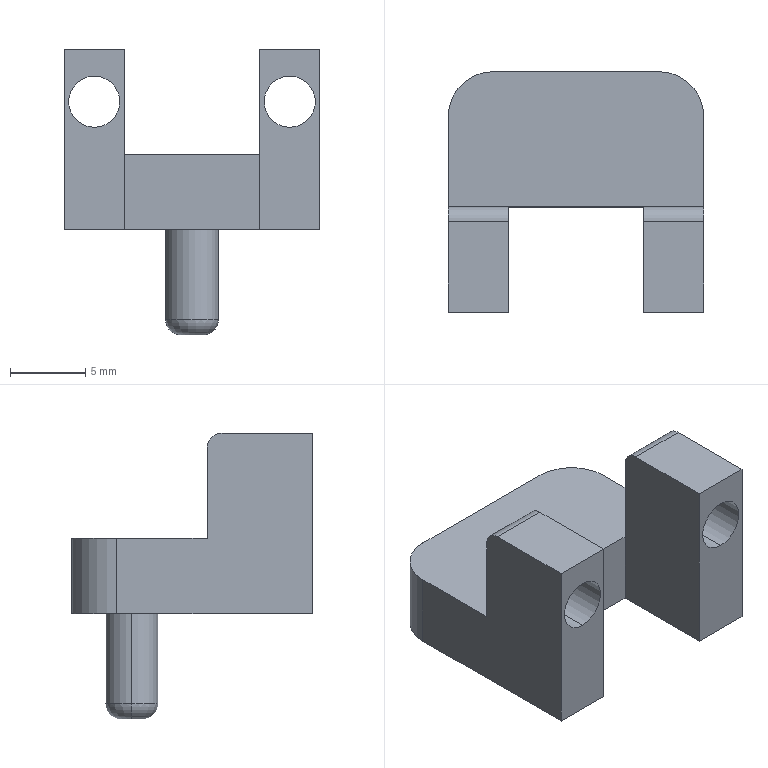Component | SolidWorks | MGL-PACK-01-00WeldedPlate1Assembly-1_MGL-PACK-01-02LocatingBlock-1 | 2 solids | 28 faces | box 17 x 16 x 19 mm | volume 1354 mm3 | plane 16 | cylinder 10 | torus 2 | commonest cylinder face diameters 3.4 x4 3.5 x2 6 x2 2 x2
STEP:
#1=COLOUR_RGB('',0.7922,0.8196,0.9333);
#2=FILL_AREA_STYLE_COLOUR('',#1);
#3=FILL_AREA_STYLE('',(#2));
#4=SURFACE_STYLE_FILL_AREA(#3);
#5=SURFACE_SIDE_STYLE('',(#4));
#6=SURFACE_STYLE_USAGE(.BOTH.,#5);
#7=PRESENTATION_STYLE_ASSIGNMENT((#6));
#8=CARTESIAN_POINT('',(-6.341,1.831,0.2677));
#9=VERTEX_POINT('',#8);
#10=CARTESIAN_POINT('',(-6.341,1.831,0.4016));
#11=VERTEX_POINT('',#10);
#12=CARTESIAN_POINT('',(-6.341,1.831,0.3346));
#13=DIRECTION('',(-0.,1.,0.));
#14=DIRECTION('',(-1.,0.,0.));
#15=AXIS2_PLACEMENT_3D('',#12,#13,#14);
#16=CIRCLE('',#15,0.06693);
#17=EDGE_CURVE('',#9,#11,#16,.T.);
#18=ORIENTED_EDGE('',*,*,#17,.F.);
#19=CARTESIAN_POINT('',(-6.341,2.106,0.2677));
#20=VERTEX_POINT('',#19);
#21=CARTESIAN_POINT('',(-6.341,2.106,0.2677));
#22=DIRECTION('',(0.,1.,0.));
#23=VECTOR('',#22,39.37);
#24=LINE('',#21,#23);
#25=EDGE_CURVE('',#9,#20,#24,.T.);
#26=ORIENTED_EDGE('',*,*,#25,.T.);
#27=CARTESIAN_POINT('',(-6.341,2.106,0.4016));
#28=VERTEX_POINT('',#27);
#29=CARTESIAN_POINT('',(-6.341,2.106,0.3346));
#30=DIRECTION('',(0.,1.,0.));
#31=DIRECTION('',(0.,0.,1.));
#32=AXIS2_PLACEMENT_3D('',#29,#30,#31);
#33=CIRCLE('',#32,0.06693);
#34=EDGE_CURVE('',#20,#28,#33,.T.);
#35=ORIENTED_EDGE('',*,*,#34,.T.);
#36=CARTESIAN_POINT('',(-6.341,2.106,0.4016));
#37=DIRECTION('',(0.,1.,0.));
#38=VECTOR('',#37,39.37);
#39=LINE('',#36,#38);
#40=EDGE_CURVE('',#11,#28,#39,.T.);
#41=ORIENTED_EDGE('',*,*,#40,.F.);
#42=EDGE_LOOP('',(#18,#26,#35,#41));
#43=FACE_OUTER_BOUND('',#42,.T.);
#44=CARTESIAN_POINT('',(-6.341,2.106,0.3346));
#45=DIRECTION('',(0.,1.,0.));
#46=DIRECTION('',(0.,0.,1.));
#47=AXIS2_PLACEMENT_3D('',#44,#45,#46);
#48=CYLINDRICAL_SURFACE('',#47,0.06693);
#49=ADVANCED_FACE('',(#43),#48,.F.);
#50=CARTESIAN_POINT('',(-5.829,1.831,0.2677));
#51=VERTEX_POINT('',#50);
#52=CARTESIAN_POINT('',(-5.829,1.831,0.4016));
#53=VERTEX_POINT('',#52);
#54=CARTESIAN_POINT('',(-5.829,1.831,0.3346));
#55=DIRECTION('',(0.,1.,0.));
#56=DIRECTION('',(-1.,0.,0.));
#57=AXIS2_PLACEMENT_3D('',#54,#55,#56);
#58=CIRCLE('',#57,0.06693);
#59=EDGE_CURVE('',#51,#53,#58,.T.);
#60=ORIENTED_EDGE('',*,*,#59,.F.);
#61=CARTESIAN_POINT('',(-5.829,2.106,0.2677));
#62=VERTEX_POINT('',#61);
#63=CARTESIAN_POINT('',(-5.829,2.106,0.2677));
#64=DIRECTION('',(0.,1.,0.));
#65=VECTOR('',#64,39.37);
#66=LINE('',#63,#65);
#67=EDGE_CURVE('',#51,#62,#66,.T.);
#68=ORIENTED_EDGE('',*,*,#67,.T.);
#69=CARTESIAN_POINT('',(-5.829,2.106,0.4016));
#70=VERTEX_POINT('',#69);
#71=CARTESIAN_POINT('',(-5.829,2.106,0.3346));
#72=DIRECTION('',(0.,1.,0.));
#73=DIRECTION('',(0.,0.,1.));
#74=AXIS2_PLACEMENT_3D('',#71,#72,#73);
#75=CIRCLE('',#74,0.06693);
#76=EDGE_CURVE('',#62,#70,#75,.T.);
#77=ORIENTED_EDGE('',*,*,#76,.T.);
#78=CARTESIAN_POINT('',(-5.829,2.106,0.4016));
#79=DIRECTION('',(0.,1.,0.));
#80=VECTOR('',#79,39.37);
#81=LINE('',#78,#80);
#82=EDGE_CURVE('',#53,#70,#81,.T.);
#83=ORIENTED_EDGE('',*,*,#82,.F.);
#84=EDGE_LOOP('',(#60,#68,#77,#83));
#85=FACE_OUTER_BOUND('',#84,.T.);
#86=CARTESIAN_POINT('',(-5.829,2.106,0.3346));
#87=DIRECTION('',(0.,1.,0.));
#88=DIRECTION('',(0.,0.,1.));
#89=AXIS2_PLACEMENT_3D('',#86,#87,#88);
#90=CYLINDRICAL_SURFACE('',#89,0.06693);
#91=ADVANCED_FACE('',(#85),#90,.F.);
#92=CARTESIAN_POINT('',(-6.262,1.831,0.4724));
#93=VERTEX_POINT('',#92);
#94=CARTESIAN_POINT('',(-6.262,2.067,0.4724));
#95=VERTEX_POINT('',#94);
#96=CARTESIAN_POINT('',(-6.262,1.831,0.4724));
#97=DIRECTION('',(0.,1.,0.));
#98=VECTOR('',#97,39.37);
#99=LINE('',#96,#98);
#100=EDGE_CURVE('',#93,#95,#99,.T.);
#101=ORIENTED_EDGE('',*,*,#100,.T.);
#102=CARTESIAN_POINT('',(-6.419,2.067,0.4724));
#103=VERTEX_POINT('',#102);
#104=CARTESIAN_POINT('',(-6.419,2.067,0.4724));
#105=DIRECTION('',(-1.,-0.,0.));
#106=VECTOR('',#105,39.37);
#107=LINE('',#104,#106);
#108=EDGE_CURVE('',#95,#103,#107,.T.);
#109=ORIENTED_EDGE('',*,*,#108,.T.);
#110=CARTESIAN_POINT('',(-6.419,1.831,0.4724));
#111=VERTEX_POINT('',#110);
#112=CARTESIAN_POINT('',(-6.419,2.461,0.4724));
#113=DIRECTION('',(-0.,-1.,0.));
#114=VECTOR('',#113,39.37);
#115=LINE('',#112,#114);
#116=EDGE_CURVE('',#103,#111,#115,.T.);
#117=ORIENTED_EDGE('',*,*,#116,.T.);
#118=CARTESIAN_POINT('',(-6.419,1.831,0.4724));
#119=DIRECTION('',(1.,0.,0.));
#120=VECTOR('',#119,39.37);
#121=LINE('',#118,#120);
#122=EDGE_CURVE('',#111,#93,#121,.T.);
#123=ORIENTED_EDGE('',*,*,#122,.T.);
#124=EDGE_LOOP('',(#101,#109,#117,#123));
#125=FACE_OUTER_BOUND('',#124,.T.);
#126=CARTESIAN_POINT('',(-6.085,2.146,0.4724));
#127=DIRECTION('',(0.,0.,1.));
#128=DIRECTION('',(1.,0.,0.));
#129=AXIS2_PLACEMENT_3D('',#126,#127,#128);
#130=PLANE('',#129);
#131=ADVANCED_FACE('',(#125),#130,.T.);
#132=ORIENTED_EDGE('',*,*,#116,.F.);
#133=CARTESIAN_POINT('',(-6.419,2.106,0.4331));
#134=VERTEX_POINT('',#133);
#135=CARTESIAN_POINT('',(-6.419,2.067,0.4331));
#136=DIRECTION('',(-1.,0.,0.));
#137=DIRECTION('',(0.,1.,0.));
#138=AXIS2_PLACEMENT_3D('',#135,#136,#137);
#139=CIRCLE('',#138,0.03937);
#140=EDGE_CURVE('',#103,#134,#139,.T.);
#141=ORIENTED_EDGE('',*,*,#140,.T.);
#142=CARTESIAN_POINT('',(-6.419,2.106,0.1969));
#143=VERTEX_POINT('',#142);
#144=CARTESIAN_POINT('',(-6.419,2.106,0.1969));
#145=DIRECTION('',(0.,0.,1.));
#146=VECTOR('',#145,39.37);
#147=LINE('',#144,#146);
#148=EDGE_CURVE('',#143,#134,#147,.T.);
#149=ORIENTED_EDGE('',*,*,#148,.F.);
#150=CARTESIAN_POINT('',(-6.419,2.343,0.1969));
#151=VERTEX_POINT('',#150);
#152=CARTESIAN_POINT('',(-6.419,2.106,0.1969));
#153=DIRECTION('',(0.,-1.,0.));
#154=VECTOR('',#153,39.37);
#155=LINE('',#152,#154);
#156=EDGE_CURVE('',#151,#143,#155,.T.);
#157=ORIENTED_EDGE('',*,*,#156,.F.);
#158=CARTESIAN_POINT('',(-6.419,2.343,-0.));
#159=VERTEX_POINT('',#158);
#160=CARTESIAN_POINT('',(-6.419,2.343,0.4724));
#161=DIRECTION('',(0.,0.,-1.));
#162=VECTOR('',#161,39.37);
#163=LINE('',#160,#162);
#164=EDGE_CURVE('',#151,#159,#163,.T.);
#165=ORIENTED_EDGE('',*,*,#164,.T.);
#166=CARTESIAN_POINT('',(-6.419,1.831,-0.));
#167=VERTEX_POINT('',#166);
#168=CARTESIAN_POINT('',(-6.419,2.461,-0.));
#169=DIRECTION('',(-0.,-1.,0.));
#170=VECTOR('',#169,39.37);
#171=LINE('',#168,#170);
#172=EDGE_CURVE('',#159,#167,#171,.T.);
#173=ORIENTED_EDGE('',*,*,#172,.T.);
#174=CARTESIAN_POINT('',(-6.419,1.831,0.4724));
#175=DIRECTION('',(0.,0.,-1.));
#176=VECTOR('',#175,39.37);
#177=LINE('',#174,#176);
#178=EDGE_CURVE('',#111,#167,#177,.T.);
#179=ORIENTED_EDGE('',*,*,#178,.F.);
#180=EDGE_LOOP('',(#132,#141,#149,#157,#165,#173,#179));
#181=FACE_OUTER_BOUND('',#180,.T.);
#182=CARTESIAN_POINT('',(-6.419,2.461,0.4724));
#183=DIRECTION('',(1.,-0.,0.));
#184=DIRECTION('',(0.,1.,0.));
#185=AXIS2_PLACEMENT_3D('',#182,#183,#184);
#186=PLANE('',#185);
#187=ADVANCED_FACE('',(#181),#186,.F.);
#188=CARTESIAN_POINT('',(-6.341,1.831,0.3346));
#189=DIRECTION('',(-0.,1.,0.));
#190=DIRECTION('',(-1.,0.,0.));
#191=AXIS2_PLACEMENT_3D('',#188,#189,#190);
#192=CIRCLE('',#191,0.06693);
#193=EDGE_CURVE('',#11,#9,#192,.T.);
#194=ORIENTED_EDGE('',*,*,#193,.T.);
#195=ORIENTED_EDGE('',*,*,#17,.T.);
#196=EDGE_LOOP('',(#194,#195));
#197=FACE_BOUND('',#196,.T.);
#198=CARTESIAN_POINT('',(-6.262,1.831,-0.));
#199=VERTEX_POINT('',#198);
#200=CARTESIAN_POINT('',(-6.419,1.831,-0.));
#201=DIRECTION('',(1.,0.,0.));
#202=VECTOR('',#201,39.37);
#203=LINE('',#200,#202);
#204=EDGE_CURVE('',#167,#199,#203,.T.);
#205=ORIENTED_EDGE('',*,*,#204,.T.);
#206=CARTESIAN_POINT('',(-6.262,1.831,0.4724));
#207=DIRECTION('',(0.,0.,-1.));
#208=VECTOR('',#207,39.37);
#209=LINE('',#206,#208);
#210=EDGE_CURVE('',#93,#199,#209,.T.);
#211=ORIENTED_EDGE('',*,*,#210,.F.);
#212=ORIENTED_EDGE('',*,*,#122,.F.);
#213=ORIENTED_EDGE('',*,*,#178,.T.);
#214=EDGE_LOOP('',(#205,#211,#212,#213));
#215=FACE_OUTER_BOUND('',#214,.T.);
#216=CARTESIAN_POINT('',(-6.419,1.831,0.4724));
#217=DIRECTION('',(-0.,1.,0.));
#218=DIRECTION('',(-1.,-0.,0.));
#219=AXIS2_PLACEMENT_3D('',#216,#217,#218);
#220=PLANE('',#219);
#221=ADVANCED_FACE('',(#197,#215),#220,.F.);
#222=CARTESIAN_POINT('',(-6.262,2.106,0.4331));
#223=VERTEX_POINT('',#222);
#224=CARTESIAN_POINT('',(-6.262,2.106,0.1969));
#225=VERTEX_POINT('',#224);
#226=CARTESIAN_POINT('',(-6.262,2.106,0.4724));
#227=DIRECTION('',(0.,0.,-1.));
#228=VECTOR('',#227,39.37);
#229=LINE('',#226,#228);
#230=EDGE_CURVE('',#223,#225,#229,.T.);
#231=ORIENTED_EDGE('',*,*,#230,.F.);
#232=CARTESIAN_POINT('',(-6.262,2.067,0.4331));
#233=DIRECTION('',(1.,0.,0.));
#234=DIRECTION('',(0.,0.,1.));
#235=AXIS2_PLACEMENT_3D('',#232,#233,#234);
#236=CIRCLE('',#235,0.03937);
#237=EDGE_CURVE('',#223,#95,#236,.T.);
#238=ORIENTED_EDGE('',*,*,#237,.T.);
#239=ORIENTED_EDGE('',*,*,#100,.F.);
#240=ORIENTED_EDGE('',*,*,#210,.T.);
#241=CARTESIAN_POINT('',(-6.262,2.106,-0.));
#242=VERTEX_POINT('',#241);
#243=CARTESIAN_POINT('',(-6.262,1.831,-0.));
#244=DIRECTION('',(0.,1.,0.));
#245=VECTOR('',#244,39.37);
#246=LINE('',#243,#245);
#247=EDGE_CURVE('',#199,#242,#246,.T.);
#248=ORIENTED_EDGE('',*,*,#247,.T.);
#249=CARTESIAN_POINT('',(-6.262,2.106,0.4724));
#250=DIRECTION('',(0.,0.,-1.));
#251=VECTOR('',#250,39.37);
#252=LINE('',#249,#251);
#253=EDGE_CURVE('',#225,#242,#252,.T.);
#254=ORIENTED_EDGE('',*,*,#253,.F.);
#255=EDGE_LOOP('',(#231,#238,#239,#240,#248,#254));
#256=FACE_OUTER_BOUND('',#255,.T.);
#257=CARTESIAN_POINT('',(-6.262,1.831,0.4724));
#258=DIRECTION('',(-1.,0.,0.));
#259=DIRECTION('',(0.,0.,1.));
#260=AXIS2_PLACEMENT_3D('',#257,#258,#259);
#261=PLANE('',#260);
#262=ADVANCED_FACE('',(#256),#261,.F.);
#263=CARTESIAN_POINT('',(-5.907,2.106,0.1969));
#264=VERTEX_POINT('',#263);
#265=CARTESIAN_POINT('',(-5.907,2.106,-0.));
#266=VERTEX_POINT('',#265);
#267=CARTESIAN_POINT('',(-5.907,2.106,0.4724));
#268=DIRECTION('',(0.,0.,-1.));
#269=VECTOR('',#268,39.37);
#270=LINE('',#267,#269);
#271=EDGE_CURVE('',#264,#266,#270,.T.);
#272=ORIENTED_EDGE('',*,*,#271,.F.);
#273=CARTESIAN_POINT('',(-6.262,2.106,0.1969));
#274=DIRECTION('',(1.,0.,0.));
#275=VECTOR('',#274,39.37);
#276=LINE('',#273,#275);
#277=EDGE_CURVE('',#225,#264,#276,.T.);
#278=ORIENTED_EDGE('',*,*,#277,.F.);
#279=ORIENTED_EDGE('',*,*,#253,.T.);
#280=CARTESIAN_POINT('',(-6.262,2.106,-0.));
#281=DIRECTION('',(1.,0.,0.));
#282=VECTOR('',#281,39.37);
#283=LINE('',#280,#282);
#284=EDGE_CURVE('',#242,#266,#283,.T.);
#285=ORIENTED_EDGE('',*,*,#284,.T.);
#286=EDGE_LOOP('',(#272,#278,#279,#285));
#287=FACE_OUTER_BOUND('',#286,.T.);
#288=CARTESIAN_POINT('',(-6.262,2.106,0.4724));
#289=DIRECTION('',(0.,1.,0.));
#290=DIRECTION('',(0.,0.,1.));
#291=AXIS2_PLACEMENT_3D('',#288,#289,#290);
#292=PLANE('',#291);
#293=ADVANCED_FACE('',(#287),#292,.F.);
#294=CARTESIAN_POINT('',(-5.907,2.067,0.4724));
#295=VERTEX_POINT('',#294);
#296=CARTESIAN_POINT('',(-5.907,1.831,0.4724));
#297=VERTEX_POINT('',#296);
#298=CARTESIAN_POINT('',(-5.907,2.106,0.4724));
#299=DIRECTION('',(0.,-1.,0.));
#300=VECTOR('',#299,39.37);
#301=LINE('',#298,#300);
#302=EDGE_CURVE('',#295,#297,#301,.T.);
#303=ORIENTED_EDGE('',*,*,#302,.F.);
#304=CARTESIAN_POINT('',(-5.907,2.106,0.4331));
#305=VERTEX_POINT('',#304);
#306=CARTESIAN_POINT('',(-5.907,2.067,0.4331));
#307=DIRECTION('',(-1.,0.,0.));
#308=DIRECTION('',(0.,0.,-1.));
#309=AXIS2_PLACEMENT_3D('',#306,#307,#308);
#310=CIRCLE('',#309,0.03937);
#311=EDGE_CURVE('',#295,#305,#310,.T.);
#312=ORIENTED_EDGE('',*,*,#311,.T.);
#313=CARTESIAN_POINT('',(-5.907,2.106,0.4724));
#314=DIRECTION('',(0.,0.,-1.));
#315=VECTOR('',#314,39.37);
#316=LINE('',#313,#315);
#317=EDGE_CURVE('',#305,#264,#316,.T.);
#318=ORIENTED_EDGE('',*,*,#317,.T.);
#319=ORIENTED_EDGE('',*,*,#271,.T.);
#320=CARTESIAN_POINT('',(-5.907,1.831,-0.));
#321=VERTEX_POINT('',#320);
#322=CARTESIAN_POINT('',(-5.907,2.106,-0.));
#323=DIRECTION('',(0.,-1.,0.));
#324=VECTOR('',#323,39.37);
#325=LINE('',#322,#324);
#326=EDGE_CURVE('',#266,#321,#325,.T.);
#327=ORIENTED_EDGE('',*,*,#326,.T.);
#328=CARTESIAN_POINT('',(-5.907,1.831,0.4724));
#329=DIRECTION('',(0.,0.,-1.));
#330=VECTOR('',#329,39.37);
#331=LINE('',#328,#330);
#332=EDGE_CURVE('',#297,#321,#331,.T.);
#333=ORIENTED_EDGE('',*,*,#332,.F.);
#334=EDGE_LOOP('',(#303,#312,#318,#319,#327,#333));
#335=FACE_OUTER_BOUND('',#334,.T.);
#336=CARTESIAN_POINT('',(-5.907,2.106,0.4724));
#337=DIRECTION('',(1.,0.,0.));
#338=DIRECTION('',(0.,0.,-1.));
#339=AXIS2_PLACEMENT_3D('',#336,#337,#338);
#340=PLANE('',#339);
#341=ADVANCED_FACE('',(#335),#340,.F.);
#342=CARTESIAN_POINT('',(-5.829,1.831,0.3346));
#343=DIRECTION('',(0.,1.,0.));
#344=DIRECTION('',(-1.,0.,0.));
#345=AXIS2_PLACEMENT_3D('',#342,#343,#344);
#346=CIRCLE('',#345,0.06693);
#347=EDGE_CURVE('',#53,#51,#346,.T.);
#348=ORIENTED_EDGE('',*,*,#347,.T.);
#349=ORIENTED_EDGE('',*,*,#59,.T.);
#350=EDGE_LOOP('',(#348,#349));
#351=FACE_BOUND('',#350,.T.);
#352=CARTESIAN_POINT('',(-5.75,1.831,-0.));
#353=VERTEX_POINT('',#352);
#354=CARTESIAN_POINT('',(-5.907,1.831,-0.));
#355=DIRECTION('',(1.,-0.,0.));
#356=VECTOR('',#355,39.37);
#357=LINE('',#354,#356);
#358=EDGE_CURVE('',#321,#353,#357,.T.);
#359=ORIENTED_EDGE('',*,*,#358,.T.);
#360=CARTESIAN_POINT('',(-5.75,1.831,0.4724));
#361=VERTEX_POINT('',#360);
#362=CARTESIAN_POINT('',(-5.75,1.831,0.4724));
#363=DIRECTION('',(0.,0.,-1.));
#364=VECTOR('',#363,39.37);
#365=LINE('',#362,#364);
#366=EDGE_CURVE('',#361,#353,#365,.T.);
#367=ORIENTED_EDGE('',*,*,#366,.F.);
#368=CARTESIAN_POINT('',(-5.907,1.831,0.4724));
#369=DIRECTION('',(1.,-0.,0.));
#370=VECTOR('',#369,39.37);
#371=LINE('',#368,#370);
#372=EDGE_CURVE('',#297,#361,#371,.T.);
#373=ORIENTED_EDGE('',*,*,#372,.F.);
#374=ORIENTED_EDGE('',*,*,#332,.T.);
#375=EDGE_LOOP('',(#359,#367,#373,#374));
#376=FACE_OUTER_BOUND('',#375,.T.);
#377=CARTESIAN_POINT('',(-5.907,1.831,0.4724));
#378=DIRECTION('',(0.,1.,0.));
#379=DIRECTION('',(-1.,0.,0.));
#380=AXIS2_PLACEMENT_3D('',#377,#378,#379);
#381=PLANE('',#380);
#382=ADVANCED_FACE('',(#351,#376),#381,.F.);
#383=CARTESIAN_POINT('',(-5.75,2.106,0.1969));
#384=VERTEX_POINT('',#383);
#385=CARTESIAN_POINT('',(-5.75,2.106,0.4331));
#386=VERTEX_POINT('',#385);
#387=CARTESIAN_POINT('',(-5.75,2.106,0.1969));
#388=DIRECTION('',(0.,0.,1.));
#389=VECTOR('',#388,39.37);
#390=LINE('',#387,#389);
#391=EDGE_CURVE('',#384,#386,#390,.T.);
#392=ORIENTED_EDGE('',*,*,#391,.T.);
#393=CARTESIAN_POINT('',(-5.75,2.067,0.4724));
#394=VERTEX_POINT('',#393);
#395=CARTESIAN_POINT('',(-5.75,2.067,0.4331));
#396=DIRECTION('',(1.,-0.,0.));
#397=DIRECTION('',(0.,-1.,0.));
#398=AXIS2_PLACEMENT_3D('',#395,#396,#397);
#399=CIRCLE('',#398,0.03937);
#400=EDGE_CURVE('',#386,#394,#399,.T.);
#401=ORIENTED_EDGE('',*,*,#400,.T.);
#402=CARTESIAN_POINT('',(-5.75,2.461,0.4724));
#403=DIRECTION('',(0.,1.,0.));
#404=VECTOR('',#403,39.37);
#405=LINE('',#402,#404);
#406=EDGE_CURVE('',#361,#394,#405,.T.);
#407=ORIENTED_EDGE('',*,*,#406,.F.);
#408=ORIENTED_EDGE('',*,*,#366,.T.);
#409=CARTESIAN_POINT('',(-5.75,2.343,-0.));
#410=VERTEX_POINT('',#409);
#411=CARTESIAN_POINT('',(-5.75,2.461,-0.));
#412=DIRECTION('',(0.,1.,0.));
#413=VECTOR('',#412,39.37);
#414=LINE('',#411,#413);
#415=EDGE_CURVE('',#353,#410,#414,.T.);
#416=ORIENTED_EDGE('',*,*,#415,.T.);
#417=CARTESIAN_POINT('',(-5.75,2.343,0.1969));
#418=VERTEX_POINT('',#417);
#419=CARTESIAN_POINT('',(-5.75,2.343,0.4724));
#420=DIRECTION('',(0.,0.,1.));
#421=VECTOR('',#420,39.37);
#422=LINE('',#419,#421);
#423=EDGE_CURVE('',#410,#418,#422,.T.);
#424=ORIENTED_EDGE('',*,*,#423,.T.);
#425=CARTESIAN_POINT('',(-5.75,2.343,0.1969));
#426=DIRECTION('',(0.,1.,0.));
#427=VECTOR('',#426,39.37);
#428=LINE('',#425,#427);
#429=EDGE_CURVE('',#384,#418,#428,.T.);
#430=ORIENTED_EDGE('',*,*,#429,.F.);
#431=EDGE_LOOP('',(#392,#401,#407,#408,#416,#424,#430));
#432=FACE_OUTER_BOUND('',#431,.T.);
#433=CARTESIAN_POINT('',(-5.75,2.461,0.4724));
#434=DIRECTION('',(-1.,0.,0.));
#435=DIRECTION('',(-0.,-1.,0.));
#436=AXIS2_PLACEMENT_3D('',#433,#434,#435);
#437=PLANE('',#436);
#438=ADVANCED_FACE('',(#432),#437,.F.);
#439=CARTESIAN_POINT('',(-6.301,2.461,-0.));
#440=VERTEX_POINT('',#439);
#441=CARTESIAN_POINT('',(-6.301,2.461,0.1969));
#442=VERTEX_POINT('',#441);
#443=CARTESIAN_POINT('',(-6.301,2.461,0.4724));
#444=DIRECTION('',(0.,0.,1.));
#445=VECTOR('',#444,39.37);
#446=LINE('',#443,#445);
#447=EDGE_CURVE('',#440,#442,#446,.T.);
#448=ORIENTED_EDGE('',*,*,#447,.T.);
#449=CARTESIAN_POINT('',(-5.868,2.461,0.1969));
#450=VERTEX_POINT('',#449);
#451=CARTESIAN_POINT('',(-6.301,2.461,0.1969));
#452=DIRECTION('',(-1.,0.,0.));
#453=VECTOR('',#452,39.37);
#454=LINE('',#451,#453);
#455=EDGE_CURVE('',#450,#442,#454,.T.);
#456=ORIENTED_EDGE('',*,*,#455,.F.);
#457=CARTESIAN_POINT('',(-5.868,2.461,-0.));
#458=VERTEX_POINT('',#457);
#459=CARTESIAN_POINT('',(-5.868,2.461,0.4724));
#460=DIRECTION('',(0.,0.,-1.));
#461=VECTOR('',#460,39.37);
#462=LINE('',#459,#461);
#463=EDGE_CURVE('',#450,#458,#462,.T.);
#464=ORIENTED_EDGE('',*,*,#463,.T.);
#465=CARTESIAN_POINT('',(-6.419,2.461,-0.));
#466=DIRECTION('',(-1.,0.,0.));
#467=VECTOR('',#466,39.37);
#468=LINE('',#465,#467);
#469=EDGE_CURVE('',#458,#440,#468,.T.);
#470=ORIENTED_EDGE('',*,*,#469,.T.);
#471=EDGE_LOOP('',(#448,#456,#464,#470));
#472=FACE_OUTER_BOUND('',#471,.T.);
#473=CARTESIAN_POINT('',(-6.419,2.461,0.4724));
#474=DIRECTION('',(0.,-1.,0.));
#475=DIRECTION('',(0.,0.,-1.));
#476=AXIS2_PLACEMENT_3D('',#473,#474,#475);
#477=PLANE('',#476);
#478=ADVANCED_FACE('',(#472),#477,.F.);
#479=ORIENTED_EDGE('',*,*,#406,.T.);
#480=CARTESIAN_POINT('',(-5.907,2.067,0.4724));
#481=DIRECTION('',(-1.,-0.,0.));
#482=VECTOR('',#481,39.37);
#483=LINE('',#480,#482);
#484=EDGE_CURVE('',#394,#295,#483,.T.);
#485=ORIENTED_EDGE('',*,*,#484,.T.);
#486=ORIENTED_EDGE('',*,*,#302,.T.);
#487=ORIENTED_EDGE('',*,*,#372,.T.);
#488=EDGE_LOOP('',(#479,#485,#486,#487));
#489=FACE_OUTER_BOUND('',#488,.T.);
#490=CARTESIAN_POINT('',(-6.085,2.146,0.4724));
#491=DIRECTION('',(0.,0.,1.));
#492=DIRECTION('',(1.,0.,0.));
#493=AXIS2_PLACEMENT_3D('',#490,#491,#492);
#494=PLANE('',#493);
#495=ADVANCED_FACE('',(#489),#494,.T.);
#496=ORIENTED_EDGE('',*,*,#469,.F.);
#497=CARTESIAN_POINT('',(-5.868,2.343,-0.));
#498=DIRECTION('',(0.,0.,-1.));
#499=DIRECTION('',(1.,0.,0.));
#500=AXIS2_PLACEMENT_3D('',#497,#498,#499);
#501=CIRCLE('',#500,0.1181);
#502=EDGE_CURVE('',#458,#410,#501,.T.);
#503=ORIENTED_EDGE('',*,*,#502,.T.);
#504=ORIENTED_EDGE('',*,*,#415,.F.);
#505=ORIENTED_EDGE('',*,*,#358,.F.);
#506=ORIENTED_EDGE('',*,*,#326,.F.);
#507=ORIENTED_EDGE('',*,*,#284,.F.);
#508=ORIENTED_EDGE('',*,*,#247,.F.);
#509=ORIENTED_EDGE('',*,*,#204,.F.);
#510=ORIENTED_EDGE('',*,*,#172,.F.);
#511=CARTESIAN_POINT('',(-6.301,2.343,-0.));
#512=DIRECTION('',(0.,0.,-1.));
#513=DIRECTION('',(1.,0.,0.));
#514=AXIS2_PLACEMENT_3D('',#511,#512,#513);
#515=CIRCLE('',#514,0.1181);
#516=EDGE_CURVE('',#159,#440,#515,.T.);
#517=ORIENTED_EDGE('',*,*,#516,.T.);
#518=EDGE_LOOP('',(#496,#503,#504,#505,#506,#507,#508,#509,#510,#517));
#519=FACE_OUTER_BOUND('',#518,.T.);
#520=CARTESIAN_POINT('',(-6.085,2.146,-0.));
#521=DIRECTION('',(0.,0.,1.));
#522=DIRECTION('',(1.,0.,0.));
#523=AXIS2_PLACEMENT_3D('',#520,#521,#522);
#524=PLANE('',#523);
#525=ADVANCED_FACE('',(#519),#524,.F.);
#526=CARTESIAN_POINT('',(-5.868,2.343,0.1969));
#527=DIRECTION('',(0.,0.,1.));
#528=DIRECTION('',(-1.,0.,0.));
#529=AXIS2_PLACEMENT_3D('',#526,#527,#528);
#530=CIRCLE('',#529,0.1181);
#531=EDGE_CURVE('',#418,#450,#530,.T.);
#532=ORIENTED_EDGE('',*,*,#531,.F.);
#533=ORIENTED_EDGE('',*,*,#423,.F.);
#534=ORIENTED_EDGE('',*,*,#502,.F.);
#535=ORIENTED_EDGE('',*,*,#463,.F.);
#536=EDGE_LOOP('',(#532,#533,#534,#535));
#537=FACE_OUTER_BOUND('',#536,.T.);
#538=CARTESIAN_POINT('',(-5.868,2.343,0.4724));
#539=DIRECTION('',(0.,0.,-1.));
#540=DIRECTION('',(-1.,0.,0.));
#541=AXIS2_PLACEMENT_3D('',#538,#539,#540);
#542=CYLINDRICAL_SURFACE('',#541,0.1181);
#543=ADVANCED_FACE('',(#537),#542,.T.);
#544=CARTESIAN_POINT('',(-6.301,2.343,0.1969));
#545=DIRECTION('',(0.,0.,1.));
#546=DIRECTION('',(-1.,0.,0.));
#547=AXIS2_PLACEMENT_3D('',#544,#545,#546);
#548=CIRCLE('',#547,0.1181);
#549=EDGE_CURVE('',#442,#151,#548,.T.);
#550=ORIENTED_EDGE('',*,*,#549,.F.);
#551=ORIENTED_EDGE('',*,*,#447,.F.);
#552=ORIENTED_EDGE('',*,*,#516,.F.);
#553=ORIENTED_EDGE('',*,*,#164,.F.);
#554=EDGE_LOOP('',(#550,#551,#552,#553));
#555=FACE_OUTER_BOUND('',#554,.T.);
#556=CARTESIAN_POINT('',(-6.301,2.343,0.4724));
#557=DIRECTION('',(0.,0.,-1.));
#558=DIRECTION('',(-1.,0.,0.));
#559=AXIS2_PLACEMENT_3D('',#556,#557,#558);
#560=CYLINDRICAL_SURFACE('',#559,0.1181);
#561=ADVANCED_FACE('',(#555),#560,.T.);
#562=CARTESIAN_POINT('',(-6.341,2.106,0.3346));
#563=DIRECTION('',(0.,1.,0.));
#564=DIRECTION('',(0.,0.,1.));
#565=AXIS2_PLACEMENT_3D('',#562,#563,#564);
#566=CIRCLE('',#565,0.06693);
#567=EDGE_CURVE('',#28,#20,#566,.T.);
#568=ORIENTED_EDGE('',*,*,#567,.F.);
#569=ORIENTED_EDGE('',*,*,#34,.F.);
#570=EDGE_LOOP('',(#568,#569));
#571=FACE_BOUND('',#570,.T.);
#572=ORIENTED_EDGE('',*,*,#148,.T.);
#573=CARTESIAN_POINT('',(-6.262,2.106,0.4331));
#574=DIRECTION('',(1.,0.,0.));
#575=VECTOR('',#574,39.37);
#576=LINE('',#573,#575);
#577=EDGE_CURVE('',#134,#223,#576,.T.);
#578=ORIENTED_EDGE('',*,*,#577,.T.);
#579=ORIENTED_EDGE('',*,*,#230,.T.);
#580=CARTESIAN_POINT('',(-6.262,2.106,0.1969));
#581=DIRECTION('',(1.,0.,0.));
#582=VECTOR('',#581,39.37);
#583=LINE('',#580,#582);
#584=EDGE_CURVE('',#143,#225,#583,.T.);
#585=ORIENTED_EDGE('',*,*,#584,.F.);
#586=EDGE_LOOP('',(#572,#578,#579,#585));
#587=FACE_OUTER_BOUND('',#586,.T.);
#588=CARTESIAN_POINT('',(-5.75,2.106,0.1969));
#589=DIRECTION('',(0.,-1.,0.));
#590=DIRECTION('',(1.,0.,0.));
#591=AXIS2_PLACEMENT_3D('',#588,#589,#590);
#592=PLANE('',#591);
#593=ADVANCED_FACE('',(#571,#587),#592,.F.);
#594=CARTESIAN_POINT('',(-5.829,2.106,0.3346));
#595=DIRECTION('',(0.,1.,0.));
#596=DIRECTION('',(0.,0.,1.));
#597=AXIS2_PLACEMENT_3D('',#594,#595,#596);
#598=CIRCLE('',#597,0.06693);
#599=EDGE_CURVE('',#70,#62,#598,.T.);
#600=ORIENTED_EDGE('',*,*,#599,.F.);
#601=ORIENTED_EDGE('',*,*,#76,.F.);
#602=EDGE_LOOP('',(#600,#601));
#603=FACE_BOUND('',#602,.T.);
#604=ORIENTED_EDGE('',*,*,#317,.F.);
#605=CARTESIAN_POINT('',(-5.75,2.106,0.4331));
#606=DIRECTION('',(1.,0.,0.));
#607=VECTOR('',#606,39.37);
#608=LINE('',#605,#607);
#609=EDGE_CURVE('',#305,#386,#608,.T.);
#610=ORIENTED_EDGE('',*,*,#609,.T.);
#611=ORIENTED_EDGE('',*,*,#391,.F.);
#612=CARTESIAN_POINT('',(-6.262,2.106,0.1969));
#613=DIRECTION('',(1.,0.,0.));
#614=VECTOR('',#613,39.37);
#615=LINE('',#612,#614);
#616=EDGE_CURVE('',#264,#384,#615,.T.);
#617=ORIENTED_EDGE('',*,*,#616,.F.);
#618=EDGE_LOOP('',(#604,#610,#611,#617));
#619=FACE_OUTER_BOUND('',#618,.T.);
#620=CARTESIAN_POINT('',(-5.75,2.106,0.1969));
#621=DIRECTION('',(0.,-1.,0.));
#622=DIRECTION('',(1.,0.,0.));
#623=AXIS2_PLACEMENT_3D('',#620,#621,#622);
#624=PLANE('',#623);
#625=ADVANCED_FACE('',(#603,#619),#624,.F.);
#626=ORIENTED_EDGE('',*,*,#584,.T.);
#627=ORIENTED_EDGE('',*,*,#277,.T.);
#628=ORIENTED_EDGE('',*,*,#616,.T.);
#629=ORIENTED_EDGE('',*,*,#429,.T.);
#630=ORIENTED_EDGE('',*,*,#531,.T.);
#631=ORIENTED_EDGE('',*,*,#455,.T.);
#632=ORIENTED_EDGE('',*,*,#549,.T.);
#633=ORIENTED_EDGE('',*,*,#156,.T.);
#634=EDGE_LOOP('',(#626,#627,#628,#629,#630,#631,#632,#633));
#635=FACE_OUTER_BOUND('',#634,.T.);
#636=CARTESIAN_POINT('',(-6.301,2.343,0.1969));
#637=DIRECTION('',(0.,0.,-1.));
#638=DIRECTION('',(-1.,0.,0.));
#639=AXIS2_PLACEMENT_3D('',#636,#637,#638);
#640=PLANE('',#639);
#641=ADVANCED_FACE('',(#635),#640,.F.);
#642=ORIENTED_EDGE('',*,*,#67,.F.);
#643=ORIENTED_EDGE('',*,*,#347,.F.);
#644=ORIENTED_EDGE('',*,*,#82,.T.);
#645=ORIENTED_EDGE('',*,*,#599,.T.);
#646=EDGE_LOOP('',(#642,#643,#644,#645));
#647=FACE_OUTER_BOUND('',#646,.T.);
#648=CARTESIAN_POINT('',(-5.829,2.106,0.3346));
#649=DIRECTION('',(0.,1.,0.));
#650=DIRECTION('',(0.,0.,1.));
#651=AXIS2_PLACEMENT_3D('',#648,#649,#650);
#652=CYLINDRICAL_SURFACE('',#651,0.06693);
#653=ADVANCED_FACE('',(#647),#652,.F.);
#654=ORIENTED_EDGE('',*,*,#25,.F.);
#655=ORIENTED_EDGE('',*,*,#193,.F.);
#656=ORIENTED_EDGE('',*,*,#40,.T.);
#657=ORIENTED_EDGE('',*,*,#567,.T.);
#658=EDGE_LOOP('',(#654,#655,#656,#657));
#659=FACE_OUTER_BOUND('',#658,.T.);
#660=CARTESIAN_POINT('',(-6.341,2.106,0.3346));
#661=DIRECTION('',(0.,1.,0.));
#662=DIRECTION('',(0.,0.,1.));
#663=AXIS2_PLACEMENT_3D('',#660,#661,#662);
#664=CYLINDRICAL_SURFACE('',#663,0.06693);
#665=ADVANCED_FACE('',(#659),#664,.F.);
#666=ORIENTED_EDGE('',*,*,#311,.F.);
#667=ORIENTED_EDGE('',*,*,#484,.F.);
#668=ORIENTED_EDGE('',*,*,#400,.F.);
#669=ORIENTED_EDGE('',*,*,#609,.F.);
#670=EDGE_LOOP('',(#666,#667,#668,#669));
#671=FACE_OUTER_BOUND('',#670,.T.);
#672=CARTESIAN_POINT('',(-5.75,2.067,0.4331));
#673=DIRECTION('',(-1.,-0.,0.));
#674=DIRECTION('',(0.,-1.,0.));
#675=AXIS2_PLACEMENT_3D('',#672,#673,#674);
#676=CYLINDRICAL_SURFACE('',#675,0.03937);
#677=ADVANCED_FACE('',(#671),#676,.T.);
#678=ORIENTED_EDGE('',*,*,#140,.F.);
#679=ORIENTED_EDGE('',*,*,#108,.F.);
#680=ORIENTED_EDGE('',*,*,#237,.F.);
#681=ORIENTED_EDGE('',*,*,#577,.F.);
#682=EDGE_LOOP('',(#678,#679,#680,#681));
#683=FACE_OUTER_BOUND('',#682,.T.);
#684=CARTESIAN_POINT('',(-5.75,2.067,0.4331));
#685=DIRECTION('',(-1.,-0.,0.));
#686=DIRECTION('',(0.,-1.,0.));
#687=AXIS2_PLACEMENT_3D('',#684,#685,#686);
#688=CYLINDRICAL_SURFACE('',#687,0.03937);
#689=ADVANCED_FACE('',(#683),#688,.T.);
#690=CLOSED_SHELL('',(#49,#91,#131,#187,#221,#262,#293,#341,#382,#438,#478,#495,#525,#543,#561,#593,#625,#641,#653,#665,#677,#689));
#691=MANIFOLD_SOLID_BREP('',#690);
#692=STYLED_ITEM('',(#7),#691);
#693=PRESENTATION_LAYER_ASSIGNMENT('','',(#692));
#694=(LENGTH_UNIT()NAMED_UNIT(*)SI_UNIT($,.METRE.));
#695=LENGTH_MEASURE_WITH_UNIT(LENGTH_MEASURE(0.0254),#694);
#696=DIMENSIONAL_EXPONENTS(1.,0.,0.,0.,0.,0.,0.);
#697=(CONVERSION_BASED_UNIT('',#695)LENGTH_UNIT()NAMED_UNIT(#696));
#698=UNCERTAINTY_MEASURE_WITH_UNIT(LENGTH_MEASURE(0.00001),#697,'','');
#699=(NAMED_UNIT(*)PLANE_ANGLE_UNIT()SI_UNIT($,.RADIAN.));
#700=(NAMED_UNIT(*)SI_UNIT($,.STERADIAN.)SOLID_ANGLE_UNIT());
#701=(GEOMETRIC_REPRESENTATION_CONTEXT(3)GLOBAL_UNCERTAINTY_ASSIGNED_CONTEXT((#698))GLOBAL_UNIT_ASSIGNED_CONTEXT((#697,#699,#700))REPRESENTATION_CONTEXT('',''));
#702=MECHANICAL_DESIGN_GEOMETRIC_PRESENTATION_REPRESENTATION('',(#692),#701);
#703=COLOUR_RGB('',0.7922,0.8196,0.9333);
#704=FILL_AREA_STYLE_COLOUR('',#703);
#705=FILL_AREA_STYLE('',(#704));
#706=SURFACE_STYLE_FILL_AREA(#705);
#707=SURFACE_SIDE_STYLE('',(#706));
#708=SURFACE_STYLE_USAGE(.BOTH.,#707);
#709=PRESENTATION_STYLE_ASSIGNMENT((#708));
#710=CARTESIAN_POINT('',(-6.114,2.303,-0.2756));
#711=VERTEX_POINT('',#710);
#712=CARTESIAN_POINT('',(-6.055,2.303,-0.2756));
#713=VERTEX_POINT('',#712);
#714=CARTESIAN_POINT('',(-6.085,2.303,-0.2756));
#715=DIRECTION('',(0.,0.,-1.));
#716=DIRECTION('',(1.,0.,0.));
#717=AXIS2_PLACEMENT_3D('',#714,#715,#716);
#718=CIRCLE('',#717,0.02953);
#719=EDGE_CURVE('',#711,#713,#718,.T.);
#720=ORIENTED_EDGE('',*,*,#719,.F.);
#721=CARTESIAN_POINT('',(-6.154,2.303,-0.2362));
#722=VERTEX_POINT('',#721);
#723=CARTESIAN_POINT('',(-6.114,2.303,-0.2362));
#724=DIRECTION('',(0.,1.,0.));
#725=DIRECTION('',(-1.,0.,0.));
#726=AXIS2_PLACEMENT_3D('',#723,#724,#725);
#727=CIRCLE('',#726,0.03937);
#728=EDGE_CURVE('',#711,#722,#727,.T.);
#729=ORIENTED_EDGE('',*,*,#728,.T.);
#730=CARTESIAN_POINT('',(-6.016,2.303,-0.2362));
#731=VERTEX_POINT('',#730);
#732=CARTESIAN_POINT('',(-6.085,2.303,-0.2362));
#733=DIRECTION('',(0.,0.,1.));
#734=DIRECTION('',(1.,0.,0.));
#735=AXIS2_PLACEMENT_3D('',#732,#733,#734);
#736=CIRCLE('',#735,0.0689);
#737=EDGE_CURVE('',#731,#722,#736,.T.);
#738=ORIENTED_EDGE('',*,*,#737,.F.);
#739=CARTESIAN_POINT('',(-6.055,2.303,-0.2362));
#740=DIRECTION('',(0.,-1.,0.));
#741=DIRECTION('',(0.,0.,-1.));
#742=AXIS2_PLACEMENT_3D('',#739,#740,#741);
#743=CIRCLE('',#742,0.03937);
#744=EDGE_CURVE('',#713,#731,#743,.T.);
#745=ORIENTED_EDGE('',*,*,#744,.F.);
#746=EDGE_LOOP('',(#720,#729,#738,#745));
#747=FACE_OUTER_BOUND('',#746,.T.);
#748=CARTESIAN_POINT('',(-6.085,2.303,-0.2362));
#749=DIRECTION('',(0.,0.,1.));
#750=DIRECTION('',(1.,0.,0.));
#751=AXIS2_PLACEMENT_3D('',#748,#749,#750);
#752=TOROIDAL_SURFACE('',#751,0.02953,0.03937);
#753=ADVANCED_FACE('',(#747),#752,.T.);
#754=ORIENTED_EDGE('',*,*,#737,.T.);
#755=CARTESIAN_POINT('',(-6.154,2.303,-0.));
#756=VERTEX_POINT('',#755);
#757=CARTESIAN_POINT('',(-6.154,2.303,-0.2756));
#758=DIRECTION('',(0.,0.,1.));
#759=VECTOR('',#758,39.37);
#760=LINE('',#757,#759);
#761=EDGE_CURVE('',#722,#756,#760,.T.);
#762=ORIENTED_EDGE('',*,*,#761,.T.);
#763=CARTESIAN_POINT('',(-6.016,2.303,-0.));
#764=VERTEX_POINT('',#763);
#765=CARTESIAN_POINT('',(-6.085,2.303,-0.));
#766=DIRECTION('',(0.,0.,1.));
#767=DIRECTION('',(1.,0.,0.));
#768=AXIS2_PLACEMENT_3D('',#765,#766,#767);
#769=CIRCLE('',#768,0.0689);
#770=EDGE_CURVE('',#764,#756,#769,.T.);
#771=ORIENTED_EDGE('',*,*,#770,.F.);
#772=CARTESIAN_POINT('',(-6.016,2.303,-0.2756));
#773=DIRECTION('',(0.,0.,1.));
#774=VECTOR('',#773,39.37);
#775=LINE('',#772,#774);
#776=EDGE_CURVE('',#731,#764,#775,.T.);
#777=ORIENTED_EDGE('',*,*,#776,.F.);
#778=EDGE_LOOP('',(#754,#762,#771,#777));
#779=FACE_OUTER_BOUND('',#778,.T.);
#780=CARTESIAN_POINT('',(-6.085,2.303,-0.2756));
#781=DIRECTION('',(0.,0.,1.));
#782=DIRECTION('',(1.,0.,0.));
#783=AXIS2_PLACEMENT_3D('',#780,#781,#782);
#784=CYLINDRICAL_SURFACE('',#783,0.0689);
#785=ADVANCED_FACE('',(#779),#784,.T.);
#786=ORIENTED_EDGE('',*,*,#761,.F.);
#787=CARTESIAN_POINT('',(-6.085,2.303,-0.2362));
#788=DIRECTION('',(0.,0.,1.));
#789=DIRECTION('',(1.,0.,0.));
#790=AXIS2_PLACEMENT_3D('',#787,#788,#789);
#791=CIRCLE('',#790,0.0689);
#792=EDGE_CURVE('',#722,#731,#791,.T.);
#793=ORIENTED_EDGE('',*,*,#792,.T.);
#794=ORIENTED_EDGE('',*,*,#776,.T.);
#795=CARTESIAN_POINT('',(-6.085,2.303,-0.));
#796=DIRECTION('',(0.,0.,1.));
#797=DIRECTION('',(1.,0.,0.));
#798=AXIS2_PLACEMENT_3D('',#795,#796,#797);
#799=CIRCLE('',#798,0.0689);
#800=EDGE_CURVE('',#756,#764,#799,.T.);
#801=ORIENTED_EDGE('',*,*,#800,.F.);
#802=EDGE_LOOP('',(#786,#793,#794,#801));
#803=FACE_OUTER_BOUND('',#802,.T.);
#804=CARTESIAN_POINT('',(-6.085,2.303,-0.2756));
#805=DIRECTION('',(0.,0.,1.));
#806=DIRECTION('',(1.,0.,0.));
#807=AXIS2_PLACEMENT_3D('',#804,#805,#806);
#808=CYLINDRICAL_SURFACE('',#807,0.0689);
#809=ADVANCED_FACE('',(#803),#808,.T.);
#810=CARTESIAN_POINT('',(-6.085,2.303,-0.2756));
#811=DIRECTION('',(0.,0.,-1.));
#812=DIRECTION('',(1.,0.,0.));
#813=AXIS2_PLACEMENT_3D('',#810,#811,#812);
#814=CIRCLE('',#813,0.02953);
#815=EDGE_CURVE('',#713,#711,#814,.T.);
#816=ORIENTED_EDGE('',*,*,#815,.T.);
#817=ORIENTED_EDGE('',*,*,#719,.T.);
#818=EDGE_LOOP('',(#816,#817));
#819=FACE_OUTER_BOUND('',#818,.T.);
#820=CARTESIAN_POINT('',(-6.085,2.303,-0.2756));
#821=DIRECTION('',(0.,0.,1.));
#822=DIRECTION('',(1.,0.,0.));
#823=AXIS2_PLACEMENT_3D('',#820,#821,#822);
#824=PLANE('',#823);
#825=ADVANCED_FACE('',(#819),#824,.F.);
#826=ORIENTED_EDGE('',*,*,#770,.T.);
#827=ORIENTED_EDGE('',*,*,#800,.T.);
#828=EDGE_LOOP('',(#826,#827));
#829=FACE_OUTER_BOUND('',#828,.T.);
#830=CARTESIAN_POINT('',(-6.085,2.303,-0.));
#831=DIRECTION('',(0.,0.,1.));
#832=DIRECTION('',(1.,0.,0.));
#833=AXIS2_PLACEMENT_3D('',#830,#831,#832);
#834=PLANE('',#833);
#835=ADVANCED_FACE('',(#829),#834,.T.);
#836=ORIENTED_EDGE('',*,*,#728,.F.);
#837=ORIENTED_EDGE('',*,*,#815,.F.);
#838=ORIENTED_EDGE('',*,*,#744,.T.);
#839=ORIENTED_EDGE('',*,*,#792,.F.);
#840=EDGE_LOOP('',(#836,#837,#838,#839));
#841=FACE_OUTER_BOUND('',#840,.T.);
#842=CARTESIAN_POINT('',(-6.085,2.303,-0.2362));
#843=DIRECTION('',(0.,0.,1.));
#844=DIRECTION('',(1.,0.,0.));
#845=AXIS2_PLACEMENT_3D('',#842,#843,#844);
#846=TOROIDAL_SURFACE('',#845,0.02953,0.03937);
#847=ADVANCED_FACE('',(#841),#846,.T.);
#848=CLOSED_SHELL('',(#753,#785,#809,#825,#835,#847));
#849=MANIFOLD_SOLID_BREP('',#848);
#850=STYLED_ITEM('',(#709),#849);
#851=(LENGTH_UNIT()NAMED_UNIT(*)SI_UNIT($,.METRE.));
#852=LENGTH_MEASURE_WITH_UNIT(LENGTH_MEASURE(0.0254),#851);
#853=DIMENSIONAL_EXPONENTS(1.,0.,0.,0.,0.,0.,0.);
#854=(CONVERSION_BASED_UNIT('',#852)LENGTH_UNIT()NAMED_UNIT(#853));
#855=UNCERTAINTY_MEASURE_WITH_UNIT(LENGTH_MEASURE(0.00001),#854,'','');
#856=(NAMED_UNIT(*)PLANE_ANGLE_UNIT()SI_UNIT($,.RADIAN.));
#857=(NAMED_UNIT(*)SI_UNIT($,.STERADIAN.)SOLID_ANGLE_UNIT());
#858=(GEOMETRIC_REPRESENTATION_CONTEXT(3)GLOBAL_UNCERTAINTY_ASSIGNED_CONTEXT((#855))GLOBAL_UNIT_ASSIGNED_CONTEXT((#854,#856,#857))REPRESENTATION_CONTEXT('',''));
#859=MECHANICAL_DESIGN_GEOMETRIC_PRESENTATION_REPRESENTATION('',(#850),#858);
#860=CARTESIAN_POINT('',(0.,0.,0.));
#861=DIRECTION('',(0.,0.,1.));
#862=DIRECTION('',(1.,0.,0.));
#863=AXIS2_PLACEMENT_3D('',#860,#861,#862);
#864=(LENGTH_UNIT()NAMED_UNIT(*)SI_UNIT($,.METRE.));
#865=LENGTH_MEASURE_WITH_UNIT(LENGTH_MEASURE(0.0254),#864);
#866=DIMENSIONAL_EXPONENTS(1.,0.,0.,0.,0.,0.,0.);
#867=(CONVERSION_BASED_UNIT('',#865)LENGTH_UNIT()NAMED_UNIT(#866));
#868=UNCERTAINTY_MEASURE_WITH_UNIT(LENGTH_MEASURE(0.00001),#867,'','');
#869=(NAMED_UNIT(*)PLANE_ANGLE_UNIT()SI_UNIT($,.RADIAN.));
#870=(NAMED_UNIT(*)SI_UNIT($,.STERADIAN.)SOLID_ANGLE_UNIT());
#871=(GEOMETRIC_REPRESENTATION_CONTEXT(3)GLOBAL_UNCERTAINTY_ASSIGNED_CONTEXT((#868))GLOBAL_UNIT_ASSIGNED_CONTEXT((#867,#869,#870))REPRESENTATION_CONTEXT('',''));
#872=ADVANCED_BREP_SHAPE_REPRESENTATION('',(#849,#691,#863),#871);
#873=PRESENTATION_LAYER_ASSIGNMENT('','',(#850));